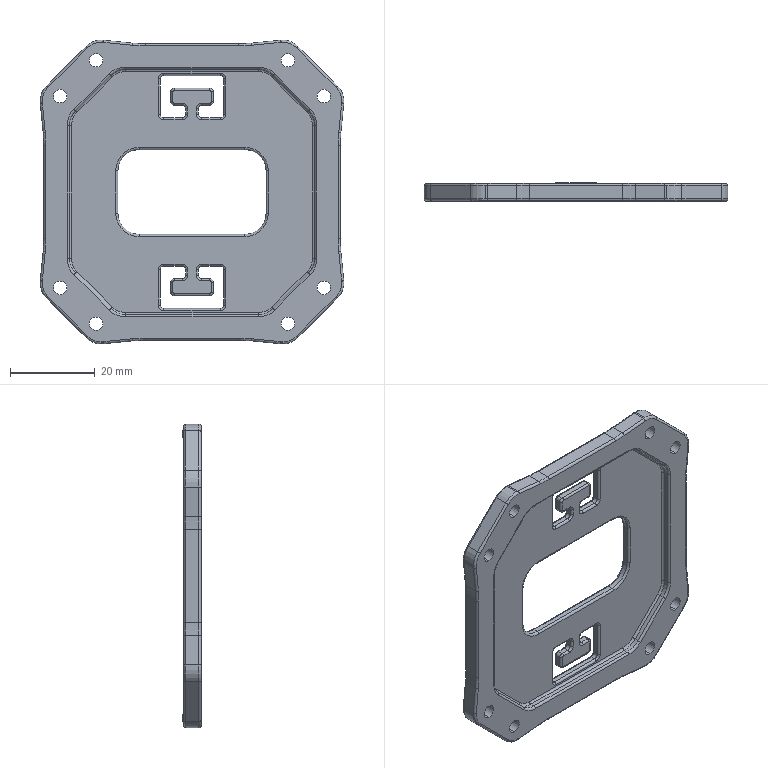Component | SolidWorks | 2.Spider top-1 | 1 solid | 731 faces | box 71.71 x 4.3 x 71.71 mm | volume 10982 mm3 | plane 299 | cylinder 174 | spline 150 | torus 108 | commonest cylinder face diameters 1 x104 1.6 x24 10 x22 3.2 x16 60 x8